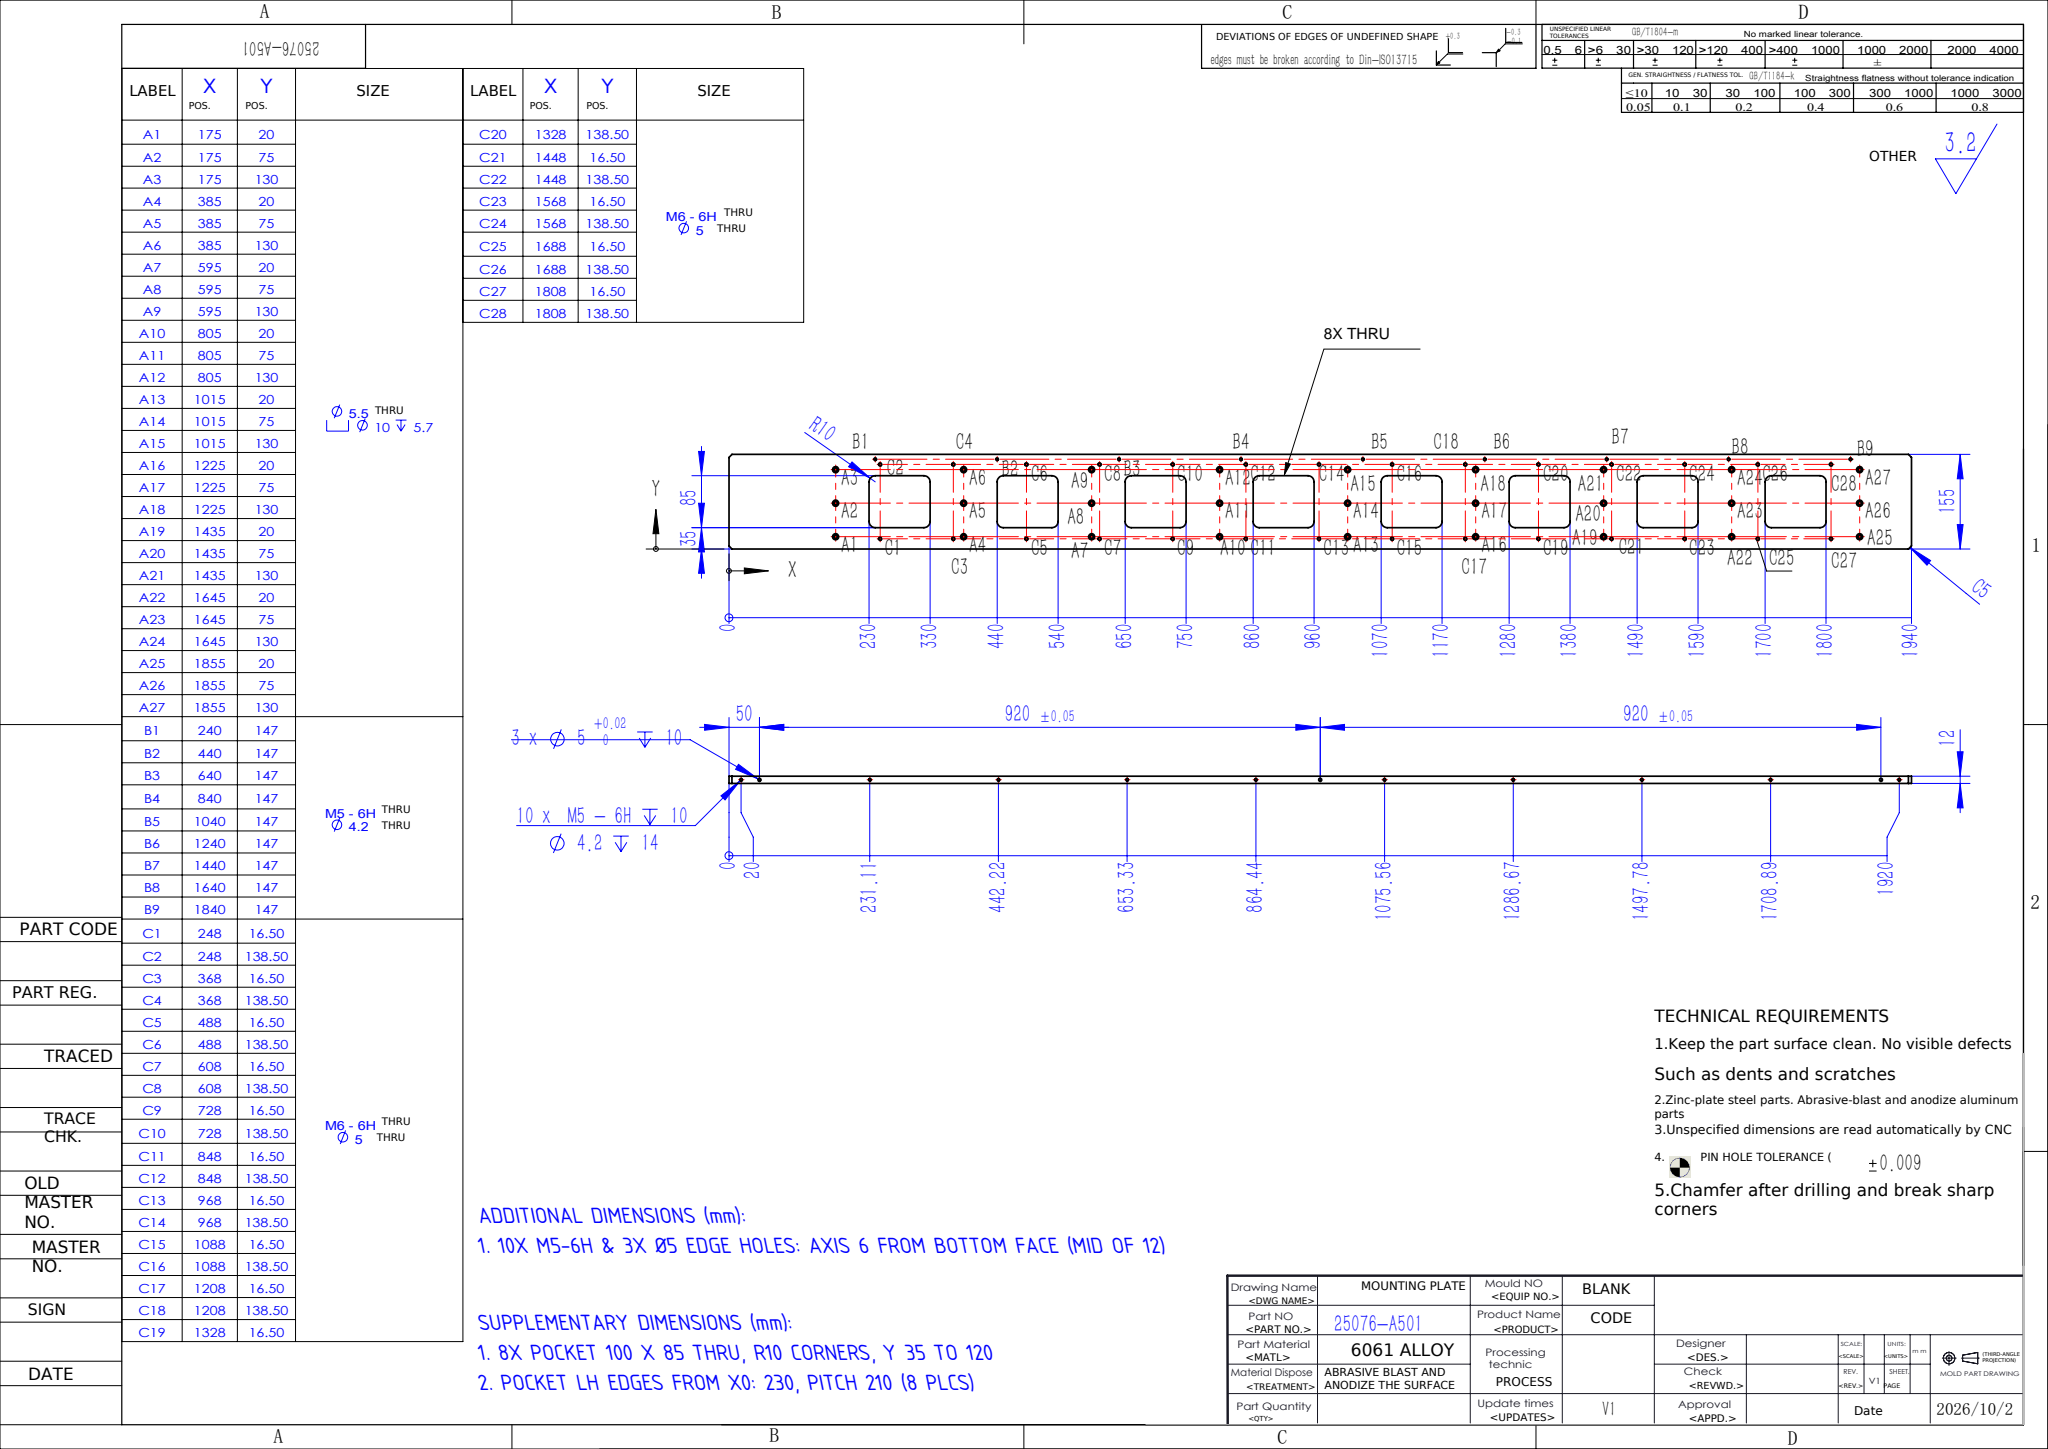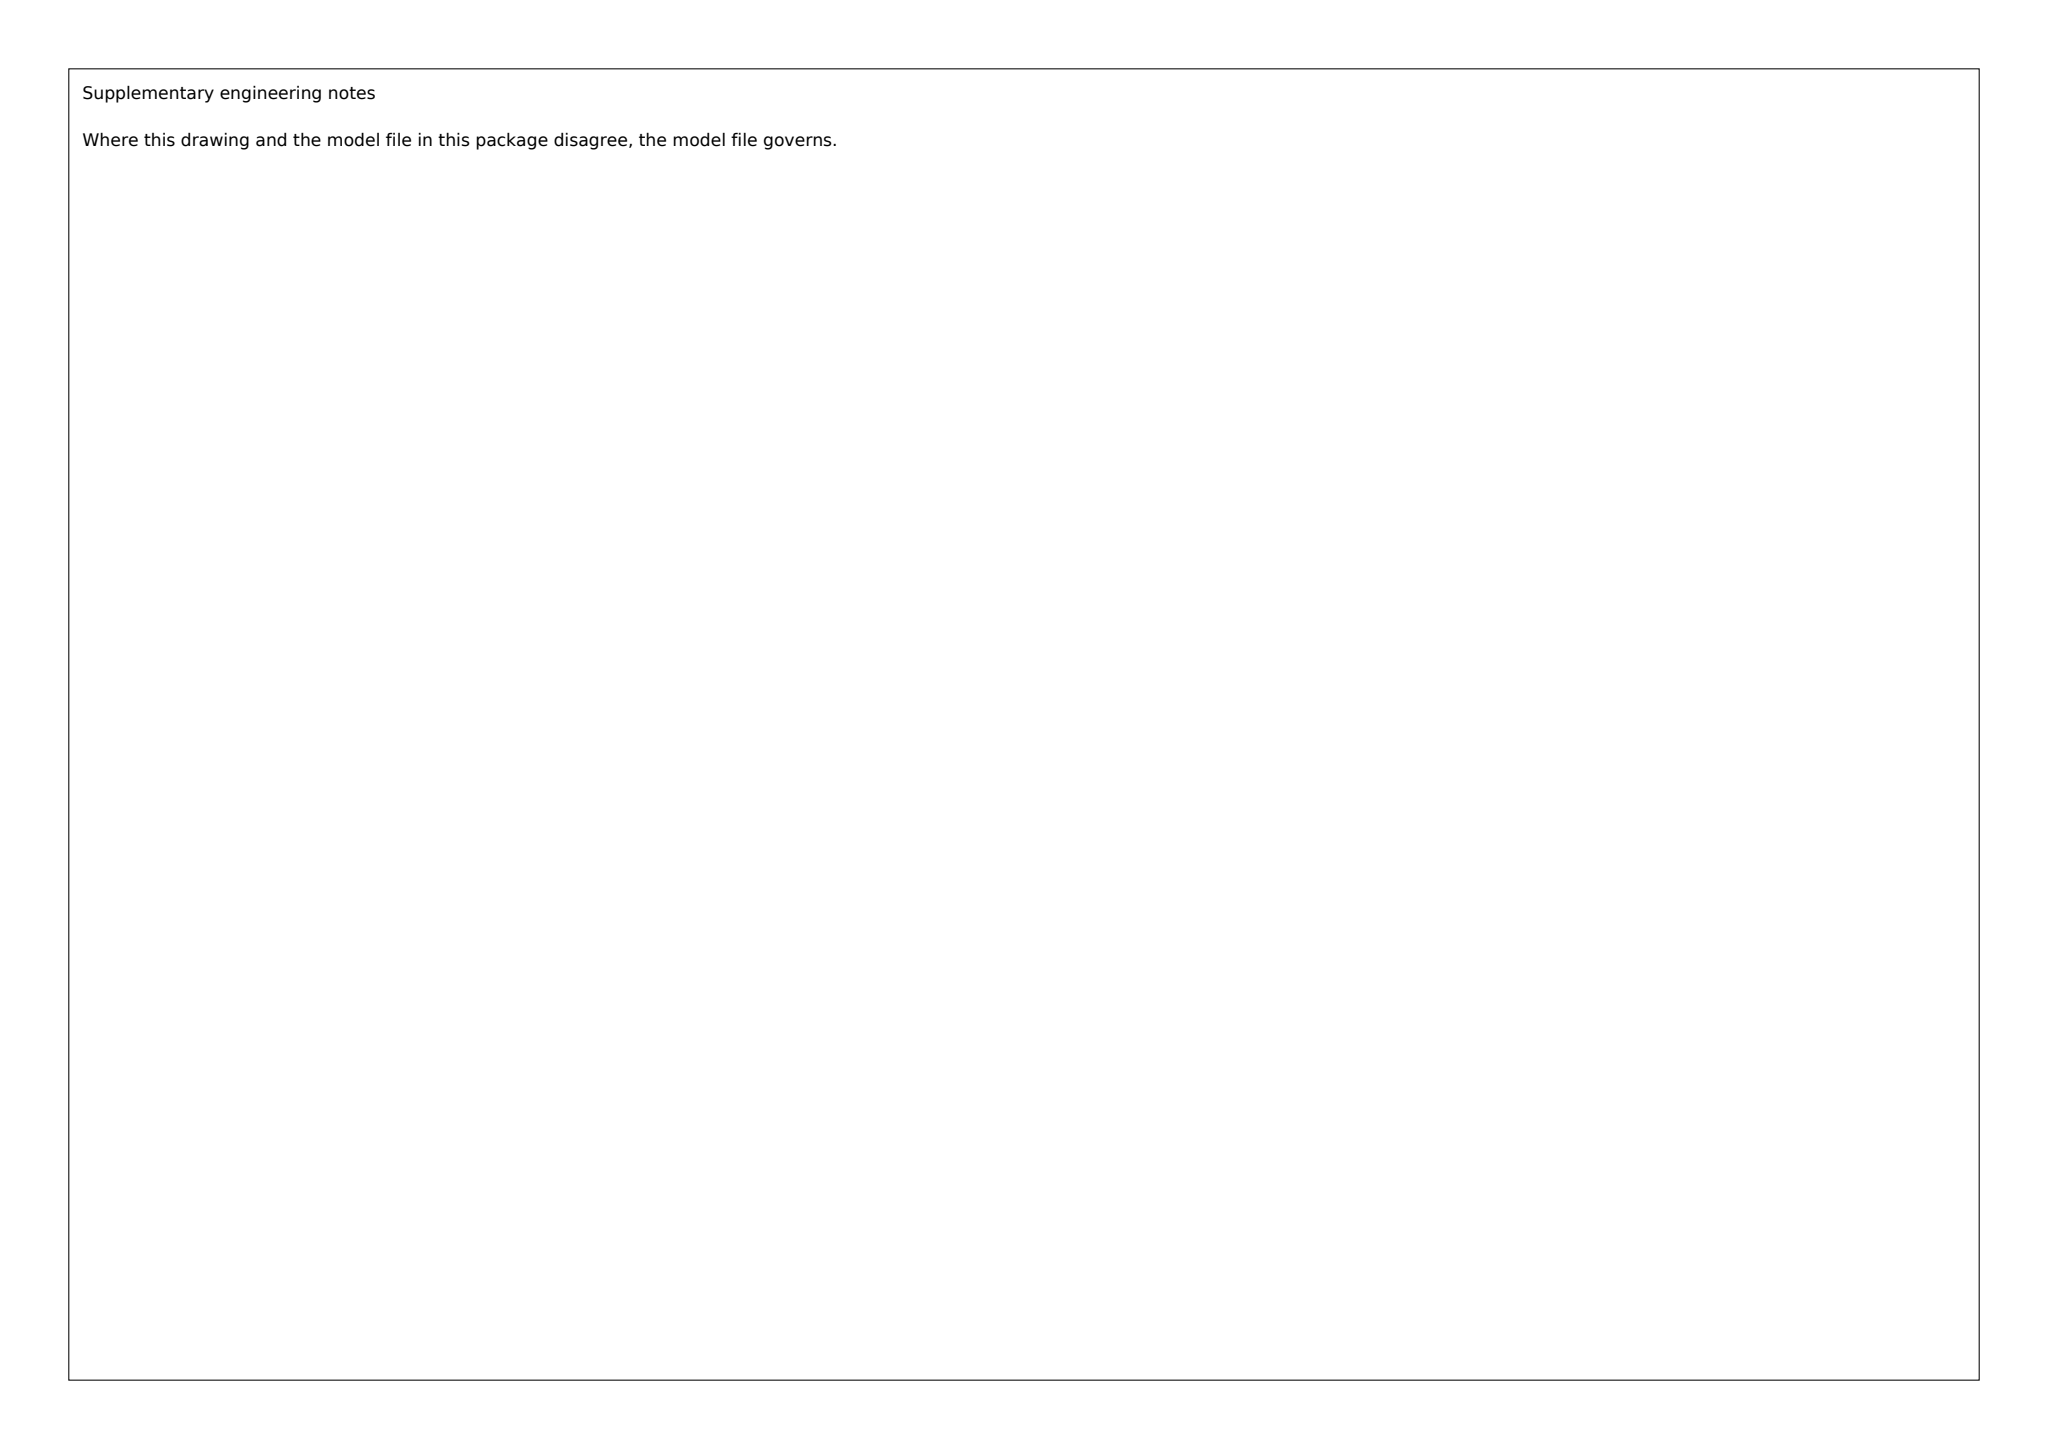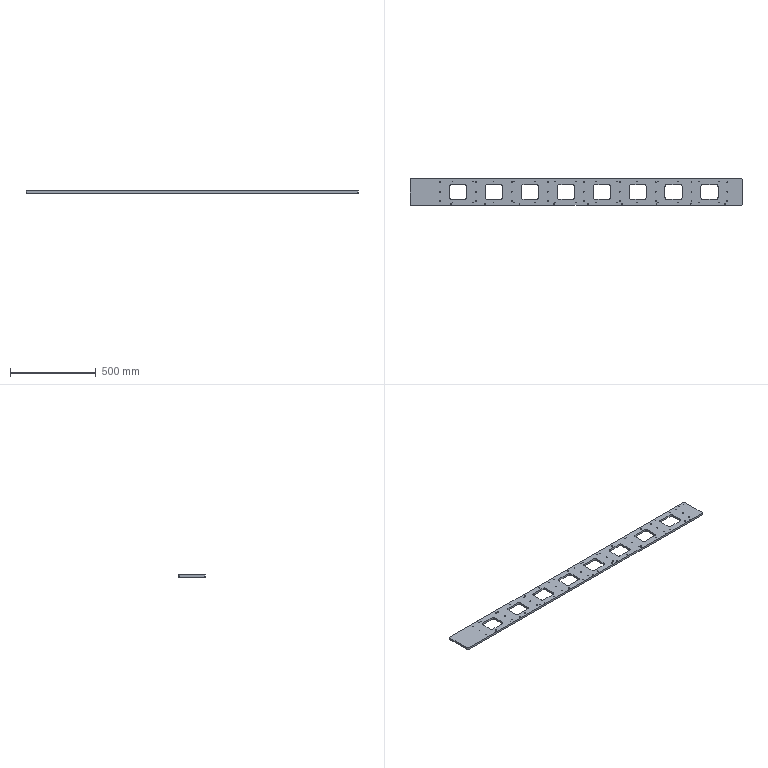Part | SolidWorks | mm | 1 solid | 335 faces | box 1940 x 155 x 12 mm | volume 2773202 mm3 | cylinder 240 | plane 69 | cone 26 | commonest cylinder face diameters 5 x62 10 x54 5.5 x54 4.2 x38 20 x32
build123d program:
from build123d import *

# Parameters (mm, degrees)
SKETCH1_W                                         = 1940
SKETCH1_H                                         = 155
BOSS_EXTRUDE1_DEPTH                               = 12
M5_TAPPED_HOLE1_D                                 = 4.2
M5_TAPPED_HOLE1_DEPTH                             = 14
M5_TAPPED_HOLE1_TIP                               = 1.262
SIZE_MM_DOWEL_PIN_HOLE_3_D                        = 5
SIZE_MM_DOWEL_PIN_HOLE_3_DEPTH                    = 10
SIZE_MM_DOWEL_PIN_HOLE_3_TIP                      = 1.502
M6_TAPPED_HOLE1_D                                 = 5
HOLE_SIZE_ACCORDING_TO_TYPE_1_OF_HEXA_D           = 5.5
HOLE_SIZE_ACCORDING_TO_TYPE_1_OF_HEXA_CBORE_D     = 10
HOLE_SIZE_ACCORDING_TO_TYPE_1_OF_HEXA_CBORE_DEPTH = 5.7
CHAMFER1_SIZE                                     = 5
SKETCH14_W                                        = 100
SKETCH14_H                                        = 85
CUT_EXTRUDE1_DEPTH                                = 974.165
FILLET1_R                                         = 10
LPATTERN1_COUNT                                   = 8
LPATTERN1_PITCH                                   = 210
FILLET1_OF_LPATTERN1_R                            = 10
M5_TAPPED_HOLE2_D                                 = 4.2


with BuildPart() as part:
    # Sketch1 → Boss-Extrude1 (new body)
    with BuildSketch(Plane.XY):
        Rectangle(SKETCH1_W, SKETCH1_H)
    extrude(amount=BOSS_EXTRUDE1_DEPTH)

    # M5 Tapped Hole1
    with Locations(Plane(origin=(0, 77.5, 0), x_dir=(1, 0, 0), z_dir=(0, 1, 0))):
        with Locations((-105.556, -6), (105.556, -6), (-316.667, -6), (316.667, -6), (527.778, -6), (-527.778, -6), (-738.889, -6), (-950, -6), (738.889, -6), (950, -6)):
            Hole(M5_TAPPED_HOLE1_D / 2, depth=M5_TAPPED_HOLE1_DEPTH)
            with Locations((0, 0, -(M5_TAPPED_HOLE1_DEPTH + M5_TAPPED_HOLE1_TIP / 2))):  # 118° drill point
                Cone(0, M5_TAPPED_HOLE1_D / 2, M5_TAPPED_HOLE1_TIP, mode=Mode.SUBTRACT)

    # Size mm Dowel Pin Hole 3
    with Locations(Plane(origin=(0, 77.5, 0), x_dir=(1, 0, 0), z_dir=(0, 1, 0))):
        with Locations((920, -6), (-920, -6), (0, -6)):
            Hole(SIZE_MM_DOWEL_PIN_HOLE_3_D / 2, depth=SIZE_MM_DOWEL_PIN_HOLE_3_DEPTH)
            with Locations((0, 0, -(SIZE_MM_DOWEL_PIN_HOLE_3_DEPTH + SIZE_MM_DOWEL_PIN_HOLE_3_TIP / 2))):  # 118° drill point
                Cone(0, SIZE_MM_DOWEL_PIN_HOLE_3_D / 2, SIZE_MM_DOWEL_PIN_HOLE_3_TIP, mode=Mode.SUBTRACT)

    # M6 Tapped Hole1 (through all)
    with Locations(Plane(origin=(0, 0, 0), x_dir=(-1, 0, 0), z_dir=(0, 0, -1))):
        with Locations((722, 61), (722, -61), (602, 61), (602, -61), (482, 61), (482, -61), (362, 61), (362, -61), (242, 61), (242, -61), (122, 61), (122, -61), (2, 61), (2, -61), (-118, 61), (-118, -61), (-238, 61), (-238, -61), (-358, 61), (-358, -61), (-478, 61), (-478, -61), (-598, 61), (-598, -61), (-718, 61), (-718, -61), (-838, 61), (-838, -61)):
            Hole(M6_TAPPED_HOLE1_D / 2)

    # Hole Size _ according to_ Type 1 of Hexa (through all)
    with Locations(Plane(origin=(0, 0, 0), x_dir=(-1, 0, 0), z_dir=(0, 0, -1))):
        with Locations((-885, 57.5), (-885, 2.5), (-885, -52.5), (-675, 57.5), (-675, 2.5), (-675, -52.5), (-465, 57.5), (-465, 2.5), (-465, -52.5), (-255, 57.5), (-255, 2.5), (-255, -52.5), (-45, 57.5), (-45, 2.5), (-45, -52.5), (165, 57.5), (165, 2.5), (165, -52.5), (375, 57.5), (375, 2.5), (375, -52.5), (585, 57.5), (585, 2.5), (585, -52.5), (795, 57.5), (795, 2.5), (795, -52.5)):
            CounterBoreHole(HOLE_SIZE_ACCORDING_TO_TYPE_1_OF_HEXA_D / 2, HOLE_SIZE_ACCORDING_TO_TYPE_1_OF_HEXA_CBORE_D / 2, HOLE_SIZE_ACCORDING_TO_TYPE_1_OF_HEXA_CBORE_DEPTH)

    # Chamfer1
    chamfer1_edges = [part.edges().sort_by_distance(p)[0] for p in [
        (970, -77.5, 6),
        (-970, -77.5, 6),
        (-970, 77.5, 6),
        (970, 77.5, 6),
    ]]
    chamfer(chamfer1_edges, length=CHAMFER1_SIZE)

    # Sketch14 → Cut-Extrude1 (cut, through all)
    with BuildSketch(Plane.XY.offset(12)):
        with Locations((780, 0)):
            Rectangle(SKETCH14_W, SKETCH14_H)
    cut_extrude1 = extrude(amount=-CUT_EXTRUDE1_DEPTH, mode=Mode.SUBTRACT)

    # Fillet1
    fillet1_edges = [part.edges().sort_by_distance(p)[0] for p in [
        (830, 42.5, 6),
        (830, -42.5, 6),
        (730, -42.5, 6),
        (730, 42.5, 6),
    ]]
    fillet(fillet1_edges, radius=FILLET1_R)

    # LPattern1: Cut-Extrude1 ×8
    with Locations(*[(-i * LPATTERN1_PITCH, 0, 0) for i in range(1, LPATTERN1_COUNT)]):
        add(cut_extrude1, mode=Mode.SUBTRACT)

    # Fillet1 of LPattern1
    fillet1_of_lpattern1_edges = [part.edges().sort_by_distance(p)[0] for p in [
        (620, 42.5, 6),
        (620, -42.5, 6),
        (520, -42.5, 6),
        (520, 42.5, 6),
        (410, 42.5, 6),
        (410, -42.5, 6),
        (310, -42.5, 6),
        (310, 42.5, 6),
        (200, 42.5, 6),
        (200, -42.5, 6),
        (100, -42.5, 6),
        (100, 42.5, 6),
        (-10, 42.5, 6),
        (-10, -42.5, 6),
        (-110, -42.5, 6),
        (-110, 42.5, 6),
        (-220, 42.5, 6),
        (-220, -42.5, 6),
        (-320, -42.5, 6),
        (-320, 42.5, 6),
        (-430, 42.5, 6),
        (-430, -42.5, 6),
        (-530, -42.5, 6),
        (-530, 42.5, 6),
        (-640, 42.5, 6),
        (-640, -42.5, 6),
        (-740, -42.5, 6),
        (-740, 42.5, 6),
    ]]
    fillet(fillet1_of_lpattern1_edges, radius=FILLET1_OF_LPATTERN1_R)

    # M5 Tapped Hole2 (through all)
    with Locations(Plane.XY.offset(12)):
        with Locations((870, -69.5), (670, -69.5), (470, -69.5), (270, -69.5), (70, -69.5), (-130, -69.5), (-330, -69.5), (-530, -69.5), (-730, -69.5)):
            Hole(M5_TAPPED_HOLE2_D / 2)


solid = part.part